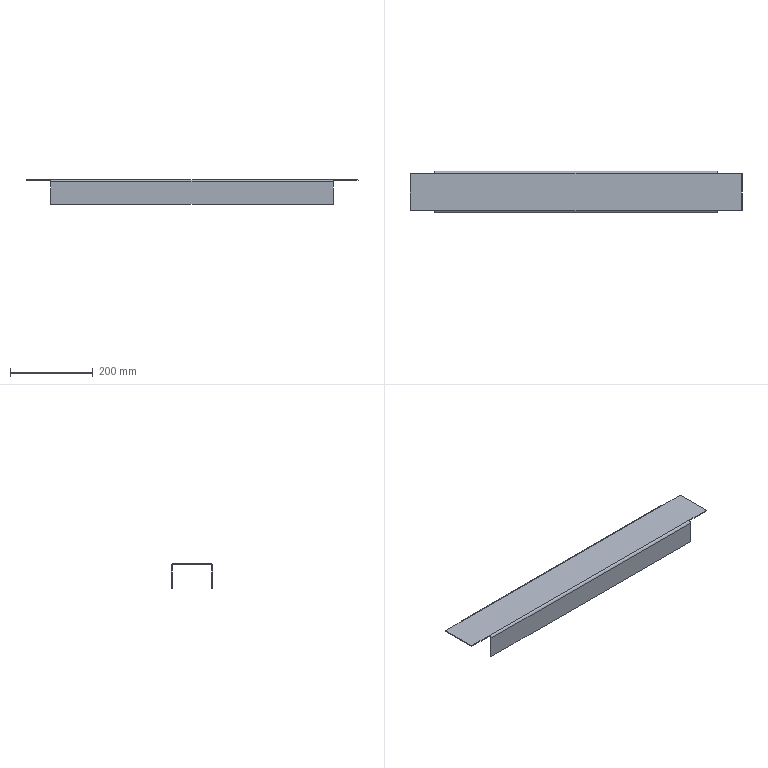Component | SolidWorks | Base-1_BaseFront-Rear-2 | 1 solid | 26 faces | box 800 x 100 x 60 mm | volume 309867 mm3 | plane 22 | cylinder 4 | commonest cylinder face diameters 7 x2 11 x2
STEP:
#1=COLOUR_RGB('',0.7922,0.8196,0.9333);
#2=FILL_AREA_STYLE_COLOUR('',#1);
#3=FILL_AREA_STYLE('',(#2));
#4=SURFACE_STYLE_FILL_AREA(#3);
#5=SURFACE_SIDE_STYLE('',(#4));
#6=SURFACE_STYLE_USAGE(.BOTH.,#5);
#7=PRESENTATION_STYLE_ASSIGNMENT((#6));
#8=CARTESIAN_POINT('',(-16.656,-4.943,13.877));
#9=VERTEX_POINT('',#8);
#10=CARTESIAN_POINT('',(-16.656,-4.943,16.023));
#11=VERTEX_POINT('',#10);
#12=CARTESIAN_POINT('',(-16.656,-4.943,16.239));
#13=DIRECTION('',(-0.,-0.,1.));
#14=VECTOR('',#13,39.37);
#15=LINE('',#12,#14);
#16=EDGE_CURVE('',#9,#11,#15,.T.);
#17=ORIENTED_EDGE('',*,*,#16,.T.);
#18=CARTESIAN_POINT('',(10.116,-4.943,16.023));
#19=VERTEX_POINT('',#18);
#20=CARTESIAN_POINT('',(-19.018,-4.943,16.023));
#21=DIRECTION('',(1.,-0.,0.));
#22=VECTOR('',#21,39.37);
#23=LINE('',#20,#22);
#24=EDGE_CURVE('',#11,#19,#23,.T.);
#25=ORIENTED_EDGE('',*,*,#24,.T.);
#26=CARTESIAN_POINT('',(10.116,-4.943,13.877));
#27=VERTEX_POINT('',#26);
#28=CARTESIAN_POINT('',(10.116,-4.943,16.239));
#29=DIRECTION('',(0.,0.,-1.));
#30=VECTOR('',#29,39.37);
#31=LINE('',#28,#30);
#32=EDGE_CURVE('',#19,#27,#31,.T.);
#33=ORIENTED_EDGE('',*,*,#32,.T.);
#34=CARTESIAN_POINT('',(-19.018,-4.943,13.877));
#35=DIRECTION('',(1.,-0.,0.));
#36=VECTOR('',#35,39.37);
#37=LINE('',#34,#36);
#38=EDGE_CURVE('',#9,#27,#37,.T.);
#39=ORIENTED_EDGE('',*,*,#38,.F.);
#40=EDGE_LOOP('',(#17,#25,#33,#39));
#41=FACE_OUTER_BOUND('',#40,.T.);
#42=CARTESIAN_POINT('',(-19.018,-4.943,16.239));
#43=DIRECTION('',(-0.,-1.,-0.));
#44=DIRECTION('',(-0.,-0.,1.));
#45=AXIS2_PLACEMENT_3D('',#42,#43,#44);
#46=PLANE('',#45);
#47=ADVANCED_FACE('',(#41),#46,.F.);
#48=CARTESIAN_POINT('',(-16.656,-5.021,13.877));
#49=VERTEX_POINT('',#48);
#50=CARTESIAN_POINT('',(10.116,-5.021,13.877));
#51=VERTEX_POINT('',#50);
#52=CARTESIAN_POINT('',(-19.018,-5.021,13.877));
#53=DIRECTION('',(1.,-0.,0.));
#54=VECTOR('',#53,39.37);
#55=LINE('',#52,#54);
#56=EDGE_CURVE('',#49,#51,#55,.T.);
#57=ORIENTED_EDGE('',*,*,#56,.F.);
#58=CARTESIAN_POINT('',(-16.656,-5.021,13.877));
#59=DIRECTION('',(0.,1.,0.));
#60=VECTOR('',#59,39.37);
#61=LINE('',#58,#60);
#62=EDGE_CURVE('',#49,#9,#61,.T.);
#63=ORIENTED_EDGE('',*,*,#62,.T.);
#64=ORIENTED_EDGE('',*,*,#38,.T.);
#65=CARTESIAN_POINT('',(10.116,-5.021,13.877));
#66=DIRECTION('',(0.,1.,0.));
#67=VECTOR('',#66,39.37);
#68=LINE('',#65,#67);
#69=EDGE_CURVE('',#51,#27,#68,.T.);
#70=ORIENTED_EDGE('',*,*,#69,.F.);
#71=EDGE_LOOP('',(#57,#63,#64,#70));
#72=FACE_OUTER_BOUND('',#71,.T.);
#73=CARTESIAN_POINT('',(-19.018,-5.021,13.877));
#74=DIRECTION('',(0.,0.,-1.));
#75=DIRECTION('',(-0.,-1.,-0.));
#76=AXIS2_PLACEMENT_3D('',#73,#74,#75);
#77=PLANE('',#76);
#78=ADVANCED_FACE('',(#72),#77,.T.);
#79=CARTESIAN_POINT('',(-16.656,-5.021,16.023));
#80=VERTEX_POINT('',#79);
#81=CARTESIAN_POINT('',(10.116,-5.021,16.023));
#82=VERTEX_POINT('',#81);
#83=CARTESIAN_POINT('',(-19.018,-5.021,16.023));
#84=DIRECTION('',(1.,-0.,0.));
#85=VECTOR('',#84,39.37);
#86=LINE('',#83,#85);
#87=EDGE_CURVE('',#80,#82,#86,.T.);
#88=ORIENTED_EDGE('',*,*,#87,.F.);
#89=CARTESIAN_POINT('',(-16.656,-5.021,16.239));
#90=DIRECTION('',(-0.,-0.,1.));
#91=VECTOR('',#90,39.37);
#92=LINE('',#89,#91);
#93=EDGE_CURVE('',#49,#80,#92,.T.);
#94=ORIENTED_EDGE('',*,*,#93,.F.);
#95=ORIENTED_EDGE('',*,*,#56,.T.);
#96=CARTESIAN_POINT('',(10.116,-5.021,16.239));
#97=DIRECTION('',(0.,0.,-1.));
#98=VECTOR('',#97,39.37);
#99=LINE('',#96,#98);
#100=EDGE_CURVE('',#82,#51,#99,.T.);
#101=ORIENTED_EDGE('',*,*,#100,.F.);
#102=EDGE_LOOP('',(#88,#94,#95,#101));
#103=FACE_OUTER_BOUND('',#102,.T.);
#104=CARTESIAN_POINT('',(-19.018,-5.021,16.239));
#105=DIRECTION('',(-0.,-1.,-0.));
#106=DIRECTION('',(-0.,-0.,1.));
#107=AXIS2_PLACEMENT_3D('',#104,#105,#106);
#108=PLANE('',#107);
#109=ADVANCED_FACE('',(#103),#108,.T.);
#110=CARTESIAN_POINT('',(-16.656,-5.159,16.16));
#111=VERTEX_POINT('',#110);
#112=CARTESIAN_POINT('',(10.116,-5.159,16.16));
#113=VERTEX_POINT('',#112);
#114=CARTESIAN_POINT('',(-19.018,-5.159,16.16));
#115=DIRECTION('',(1.,-0.,0.));
#116=VECTOR('',#115,39.37);
#117=LINE('',#114,#116);
#118=EDGE_CURVE('',#111,#113,#117,.T.);
#119=ORIENTED_EDGE('',*,*,#118,.F.);
#120=CARTESIAN_POINT('',(-16.656,-5.159,16.023));
#121=DIRECTION('',(1.,-0.,0.));
#122=DIRECTION('',(0.,0.,-1.));
#123=AXIS2_PLACEMENT_3D('',#120,#121,#122);
#124=CIRCLE('',#123,0.1378);
#125=EDGE_CURVE('',#80,#111,#124,.T.);
#126=ORIENTED_EDGE('',*,*,#125,.F.);
#127=ORIENTED_EDGE('',*,*,#87,.T.);
#128=CARTESIAN_POINT('',(10.116,-5.159,16.023));
#129=DIRECTION('',(-1.,0.,-0.));
#130=DIRECTION('',(0.,-1.,0.));
#131=AXIS2_PLACEMENT_3D('',#128,#129,#130);
#132=CIRCLE('',#131,0.1378);
#133=EDGE_CURVE('',#113,#82,#132,.T.);
#134=ORIENTED_EDGE('',*,*,#133,.F.);
#135=EDGE_LOOP('',(#119,#126,#127,#134));
#136=FACE_OUTER_BOUND('',#135,.T.);
#137=CARTESIAN_POINT('',(-19.018,-5.159,16.023));
#138=DIRECTION('',(1.,-0.,0.));
#139=DIRECTION('',(0.,0.,-1.));
#140=AXIS2_PLACEMENT_3D('',#137,#138,#139);
#141=CYLINDRICAL_SURFACE('',#140,0.1378);
#142=ADVANCED_FACE('',(#136),#141,.F.);
#143=CARTESIAN_POINT('',(-16.656,-5.159,16.239));
#144=VERTEX_POINT('',#143);
#145=CARTESIAN_POINT('',(-16.656,-5.159,16.023));
#146=DIRECTION('',(1.,-0.,0.));
#147=DIRECTION('',(0.,0.,-1.));
#148=AXIS2_PLACEMENT_3D('',#145,#146,#147);
#149=CIRCLE('',#148,0.2165);
#150=EDGE_CURVE('',#11,#144,#149,.T.);
#151=ORIENTED_EDGE('',*,*,#150,.T.);
#152=CARTESIAN_POINT('',(10.116,-5.159,16.239));
#153=VERTEX_POINT('',#152);
#154=CARTESIAN_POINT('',(-19.018,-5.159,16.239));
#155=DIRECTION('',(1.,-0.,0.));
#156=VECTOR('',#155,39.37);
#157=LINE('',#154,#156);
#158=EDGE_CURVE('',#144,#153,#157,.T.);
#159=ORIENTED_EDGE('',*,*,#158,.T.);
#160=CARTESIAN_POINT('',(10.116,-5.159,16.023));
#161=DIRECTION('',(-1.,0.,-0.));
#162=DIRECTION('',(0.,0.,-1.));
#163=AXIS2_PLACEMENT_3D('',#160,#161,#162);
#164=CIRCLE('',#163,0.2165);
#165=EDGE_CURVE('',#153,#19,#164,.T.);
#166=ORIENTED_EDGE('',*,*,#165,.T.);
#167=ORIENTED_EDGE('',*,*,#24,.F.);
#168=EDGE_LOOP('',(#151,#159,#166,#167));
#169=FACE_OUTER_BOUND('',#168,.T.);
#170=CARTESIAN_POINT('',(-19.018,-5.159,16.023));
#171=DIRECTION('',(1.,-0.,0.));
#172=DIRECTION('',(0.,0.,-1.));
#173=AXIS2_PLACEMENT_3D('',#170,#171,#172);
#174=CYLINDRICAL_SURFACE('',#173,0.2165);
#175=ADVANCED_FACE('',(#169),#174,.T.);
#176=CARTESIAN_POINT('',(-16.656,-8.663,16.16));
#177=VERTEX_POINT('',#176);
#178=CARTESIAN_POINT('',(10.116,-8.663,16.16));
#179=VERTEX_POINT('',#178);
#180=CARTESIAN_POINT('',(-19.018,-8.663,16.16));
#181=DIRECTION('',(1.,-0.,0.));
#182=VECTOR('',#181,39.37);
#183=LINE('',#180,#182);
#184=EDGE_CURVE('',#177,#179,#183,.T.);
#185=ORIENTED_EDGE('',*,*,#184,.T.);
#186=CARTESIAN_POINT('',(10.116,-8.801,16.023));
#187=VERTEX_POINT('',#186);
#188=CARTESIAN_POINT('',(10.116,-8.663,16.023));
#189=DIRECTION('',(-1.,0.,-0.));
#190=DIRECTION('',(0.,-1.,0.));
#191=AXIS2_PLACEMENT_3D('',#188,#189,#190);
#192=CIRCLE('',#191,0.1378);
#193=EDGE_CURVE('',#187,#179,#192,.T.);
#194=ORIENTED_EDGE('',*,*,#193,.F.);
#195=CARTESIAN_POINT('',(-16.656,-8.801,16.023));
#196=VERTEX_POINT('',#195);
#197=CARTESIAN_POINT('',(-19.018,-8.801,16.023));
#198=DIRECTION('',(1.,-0.,0.));
#199=VECTOR('',#198,39.37);
#200=LINE('',#197,#199);
#201=EDGE_CURVE('',#196,#187,#200,.T.);
#202=ORIENTED_EDGE('',*,*,#201,.F.);
#203=CARTESIAN_POINT('',(-16.656,-8.663,16.023));
#204=DIRECTION('',(1.,-0.,0.));
#205=DIRECTION('',(0.,0.,-1.));
#206=AXIS2_PLACEMENT_3D('',#203,#204,#205);
#207=CIRCLE('',#206,0.1378);
#208=EDGE_CURVE('',#177,#196,#207,.T.);
#209=ORIENTED_EDGE('',*,*,#208,.F.);
#210=EDGE_LOOP('',(#185,#194,#202,#209));
#211=FACE_OUTER_BOUND('',#210,.T.);
#212=CARTESIAN_POINT('',(-19.018,-8.663,16.023));
#213=DIRECTION('',(1.,-0.,0.));
#214=DIRECTION('',(0.,0.,-1.));
#215=AXIS2_PLACEMENT_3D('',#212,#213,#214);
#216=CYLINDRICAL_SURFACE('',#215,0.1378);
#217=ADVANCED_FACE('',(#211),#216,.F.);
#218=ORIENTED_EDGE('',*,*,#201,.T.);
#219=CARTESIAN_POINT('',(10.116,-8.801,13.877));
#220=VERTEX_POINT('',#219);
#221=CARTESIAN_POINT('',(10.116,-8.801,13.877));
#222=DIRECTION('',(-0.,-0.,1.));
#223=VECTOR('',#222,39.37);
#224=LINE('',#221,#223);
#225=EDGE_CURVE('',#220,#187,#224,.T.);
#226=ORIENTED_EDGE('',*,*,#225,.F.);
#227=CARTESIAN_POINT('',(-16.656,-8.801,13.877));
#228=VERTEX_POINT('',#227);
#229=CARTESIAN_POINT('',(-19.018,-8.801,13.877));
#230=DIRECTION('',(1.,-0.,0.));
#231=VECTOR('',#230,39.37);
#232=LINE('',#229,#231);
#233=EDGE_CURVE('',#228,#220,#232,.T.);
#234=ORIENTED_EDGE('',*,*,#233,.F.);
#235=CARTESIAN_POINT('',(-16.656,-8.801,13.877));
#236=DIRECTION('',(0.,0.,-1.));
#237=VECTOR('',#236,39.37);
#238=LINE('',#235,#237);
#239=EDGE_CURVE('',#196,#228,#238,.T.);
#240=ORIENTED_EDGE('',*,*,#239,.F.);
#241=EDGE_LOOP('',(#218,#226,#234,#240));
#242=FACE_OUTER_BOUND('',#241,.T.);
#243=CARTESIAN_POINT('',(-19.018,-8.801,13.877));
#244=DIRECTION('',(0.,1.,0.));
#245=DIRECTION('',(0.,0.,-1.));
#246=AXIS2_PLACEMENT_3D('',#243,#244,#245);
#247=PLANE('',#246);
#248=ADVANCED_FACE('',(#242),#247,.T.);
#249=ORIENTED_EDGE('',*,*,#233,.T.);
#250=CARTESIAN_POINT('',(10.116,-8.88,13.877));
#251=VERTEX_POINT('',#250);
#252=CARTESIAN_POINT('',(10.116,-8.801,13.877));
#253=DIRECTION('',(-0.,-1.,-0.));
#254=VECTOR('',#253,39.37);
#255=LINE('',#252,#254);
#256=EDGE_CURVE('',#220,#251,#255,.T.);
#257=ORIENTED_EDGE('',*,*,#256,.T.);
#258=CARTESIAN_POINT('',(-16.656,-8.88,13.877));
#259=VERTEX_POINT('',#258);
#260=CARTESIAN_POINT('',(-19.018,-8.88,13.877));
#261=DIRECTION('',(1.,-0.,0.));
#262=VECTOR('',#261,39.37);
#263=LINE('',#260,#262);
#264=EDGE_CURVE('',#259,#251,#263,.T.);
#265=ORIENTED_EDGE('',*,*,#264,.F.);
#266=CARTESIAN_POINT('',(-16.656,-8.88,13.877));
#267=DIRECTION('',(0.,1.,0.));
#268=VECTOR('',#267,39.37);
#269=LINE('',#266,#268);
#270=EDGE_CURVE('',#259,#228,#269,.T.);
#271=ORIENTED_EDGE('',*,*,#270,.T.);
#272=EDGE_LOOP('',(#249,#257,#265,#271));
#273=FACE_OUTER_BOUND('',#272,.T.);
#274=CARTESIAN_POINT('',(-19.018,-8.88,13.877));
#275=DIRECTION('',(0.,0.,-1.));
#276=DIRECTION('',(-0.,-1.,-0.));
#277=AXIS2_PLACEMENT_3D('',#274,#275,#276);
#278=PLANE('',#277);
#279=ADVANCED_FACE('',(#273),#278,.T.);
#280=CARTESIAN_POINT('',(10.116,-8.88,16.023));
#281=VERTEX_POINT('',#280);
#282=CARTESIAN_POINT('',(10.116,-8.88,13.877));
#283=DIRECTION('',(-0.,-0.,1.));
#284=VECTOR('',#283,39.37);
#285=LINE('',#282,#284);
#286=EDGE_CURVE('',#251,#281,#285,.T.);
#287=ORIENTED_EDGE('',*,*,#286,.T.);
#288=CARTESIAN_POINT('',(-16.656,-8.88,16.023));
#289=VERTEX_POINT('',#288);
#290=CARTESIAN_POINT('',(-19.018,-8.88,16.023));
#291=DIRECTION('',(1.,-0.,0.));
#292=VECTOR('',#291,39.37);
#293=LINE('',#290,#292);
#294=EDGE_CURVE('',#289,#281,#293,.T.);
#295=ORIENTED_EDGE('',*,*,#294,.F.);
#296=CARTESIAN_POINT('',(-16.656,-8.88,20.752));
#297=DIRECTION('',(0.,0.,-1.));
#298=VECTOR('',#297,39.37);
#299=LINE('',#296,#298);
#300=EDGE_CURVE('',#289,#259,#299,.T.);
#301=ORIENTED_EDGE('',*,*,#300,.T.);
#302=ORIENTED_EDGE('',*,*,#264,.T.);
#303=EDGE_LOOP('',(#287,#295,#301,#302));
#304=FACE_OUTER_BOUND('',#303,.T.);
#305=CARTESIAN_POINT('',(-19.018,-8.88,13.877));
#306=DIRECTION('',(0.,1.,0.));
#307=DIRECTION('',(0.,0.,-1.));
#308=AXIS2_PLACEMENT_3D('',#305,#306,#307);
#309=PLANE('',#308);
#310=ADVANCED_FACE('',(#304),#309,.F.);
#311=CARTESIAN_POINT('',(10.116,-8.663,16.239));
#312=VERTEX_POINT('',#311);
#313=CARTESIAN_POINT('',(10.116,-8.663,16.023));
#314=DIRECTION('',(-1.,0.,-0.));
#315=DIRECTION('',(0.,0.,-1.));
#316=AXIS2_PLACEMENT_3D('',#313,#314,#315);
#317=CIRCLE('',#316,0.2165);
#318=EDGE_CURVE('',#281,#312,#317,.T.);
#319=ORIENTED_EDGE('',*,*,#318,.T.);
#320=CARTESIAN_POINT('',(-16.656,-8.663,16.239));
#321=VERTEX_POINT('',#320);
#322=CARTESIAN_POINT('',(-19.018,-8.663,16.239));
#323=DIRECTION('',(1.,-0.,0.));
#324=VECTOR('',#323,39.37);
#325=LINE('',#322,#324);
#326=EDGE_CURVE('',#321,#312,#325,.T.);
#327=ORIENTED_EDGE('',*,*,#326,.F.);
#328=CARTESIAN_POINT('',(-16.656,-8.663,16.023));
#329=DIRECTION('',(1.,-0.,0.));
#330=DIRECTION('',(0.,0.,-1.));
#331=AXIS2_PLACEMENT_3D('',#328,#329,#330);
#332=CIRCLE('',#331,0.2165);
#333=EDGE_CURVE('',#321,#289,#332,.T.);
#334=ORIENTED_EDGE('',*,*,#333,.T.);
#335=ORIENTED_EDGE('',*,*,#294,.T.);
#336=EDGE_LOOP('',(#319,#327,#334,#335));
#337=FACE_OUTER_BOUND('',#336,.T.);
#338=CARTESIAN_POINT('',(-19.018,-8.663,16.023));
#339=DIRECTION('',(1.,-0.,0.));
#340=DIRECTION('',(0.,0.,-1.));
#341=AXIS2_PLACEMENT_3D('',#338,#339,#340);
#342=CYLINDRICAL_SURFACE('',#341,0.2165);
#343=ADVANCED_FACE('',(#337),#342,.T.);
#344=CARTESIAN_POINT('',(12.478,-8.663,16.239));
#345=VERTEX_POINT('',#344);
#346=CARTESIAN_POINT('',(12.478,-5.159,16.239));
#347=VERTEX_POINT('',#346);
#348=CARTESIAN_POINT('',(12.478,-8.88,16.239));
#349=DIRECTION('',(0.,1.,0.));
#350=VECTOR('',#349,39.37);
#351=LINE('',#348,#350);
#352=EDGE_CURVE('',#345,#347,#351,.T.);
#353=ORIENTED_EDGE('',*,*,#352,.F.);
#354=CARTESIAN_POINT('',(12.478,-8.663,16.16));
#355=VERTEX_POINT('',#354);
#356=CARTESIAN_POINT('',(12.478,-8.663,16.239));
#357=DIRECTION('',(0.,0.,-1.));
#358=VECTOR('',#357,39.37);
#359=LINE('',#356,#358);
#360=EDGE_CURVE('',#345,#355,#359,.T.);
#361=ORIENTED_EDGE('',*,*,#360,.T.);
#362=CARTESIAN_POINT('',(12.478,-5.159,16.16));
#363=VERTEX_POINT('',#362);
#364=CARTESIAN_POINT('',(12.478,-8.88,16.16));
#365=DIRECTION('',(0.,1.,0.));
#366=VECTOR('',#365,39.37);
#367=LINE('',#364,#366);
#368=EDGE_CURVE('',#355,#363,#367,.T.);
#369=ORIENTED_EDGE('',*,*,#368,.T.);
#370=CARTESIAN_POINT('',(12.478,-5.159,16.16));
#371=DIRECTION('',(-0.,-0.,1.));
#372=VECTOR('',#371,39.37);
#373=LINE('',#370,#372);
#374=EDGE_CURVE('',#363,#347,#373,.T.);
#375=ORIENTED_EDGE('',*,*,#374,.T.);
#376=EDGE_LOOP('',(#353,#361,#369,#375));
#377=FACE_OUTER_BOUND('',#376,.T.);
#378=CARTESIAN_POINT('',(12.478,-8.801,16.023));
#379=DIRECTION('',(1.,-0.,0.));
#380=DIRECTION('',(0.,0.,-1.));
#381=AXIS2_PLACEMENT_3D('',#378,#379,#380);
#382=PLANE('',#381);
#383=ADVANCED_FACE('',(#377),#382,.T.);
#384=CARTESIAN_POINT('',(-19.018,-8.663,16.239));
#385=VERTEX_POINT('',#384);
#386=CARTESIAN_POINT('',(-19.018,-5.159,16.239));
#387=VERTEX_POINT('',#386);
#388=CARTESIAN_POINT('',(-19.018,-8.88,16.239));
#389=DIRECTION('',(0.,1.,0.));
#390=VECTOR('',#389,39.37);
#391=LINE('',#388,#390);
#392=EDGE_CURVE('',#385,#387,#391,.T.);
#393=ORIENTED_EDGE('',*,*,#392,.T.);
#394=CARTESIAN_POINT('',(-19.018,-5.159,16.16));
#395=VERTEX_POINT('',#394);
#396=CARTESIAN_POINT('',(-19.018,-5.159,16.239));
#397=DIRECTION('',(0.,0.,-1.));
#398=VECTOR('',#397,39.37);
#399=LINE('',#396,#398);
#400=EDGE_CURVE('',#387,#395,#399,.T.);
#401=ORIENTED_EDGE('',*,*,#400,.T.);
#402=CARTESIAN_POINT('',(-19.018,-8.663,16.16));
#403=VERTEX_POINT('',#402);
#404=CARTESIAN_POINT('',(-19.018,-8.88,16.16));
#405=DIRECTION('',(0.,1.,0.));
#406=VECTOR('',#405,39.37);
#407=LINE('',#404,#406);
#408=EDGE_CURVE('',#403,#395,#407,.T.);
#409=ORIENTED_EDGE('',*,*,#408,.F.);
#410=CARTESIAN_POINT('',(-19.018,-8.663,16.16));
#411=DIRECTION('',(-0.,-0.,1.));
#412=VECTOR('',#411,39.37);
#413=LINE('',#410,#412);
#414=EDGE_CURVE('',#403,#385,#413,.T.);
#415=ORIENTED_EDGE('',*,*,#414,.T.);
#416=EDGE_LOOP('',(#393,#401,#409,#415));
#417=FACE_OUTER_BOUND('',#416,.T.);
#418=CARTESIAN_POINT('',(-19.018,-5.021,16.023));
#419=DIRECTION('',(-1.,0.,-0.));
#420=DIRECTION('',(-0.,-0.,1.));
#421=AXIS2_PLACEMENT_3D('',#418,#419,#420);
#422=PLANE('',#421);
#423=ADVANCED_FACE('',(#417),#422,.T.);
#424=ORIENTED_EDGE('',*,*,#368,.F.);
#425=CARTESIAN_POINT('',(-19.018,-8.663,16.16));
#426=DIRECTION('',(1.,-0.,0.));
#427=VECTOR('',#426,39.37);
#428=LINE('',#425,#427);
#429=EDGE_CURVE('',#179,#355,#428,.T.);
#430=ORIENTED_EDGE('',*,*,#429,.F.);
#431=ORIENTED_EDGE('',*,*,#184,.F.);
#432=CARTESIAN_POINT('',(-19.018,-8.663,16.16));
#433=DIRECTION('',(1.,-0.,0.));
#434=VECTOR('',#433,39.37);
#435=LINE('',#432,#434);
#436=EDGE_CURVE('',#403,#177,#435,.T.);
#437=ORIENTED_EDGE('',*,*,#436,.F.);
#438=ORIENTED_EDGE('',*,*,#408,.T.);
#439=CARTESIAN_POINT('',(-19.018,-5.159,16.16));
#440=DIRECTION('',(1.,-0.,0.));
#441=VECTOR('',#440,39.37);
#442=LINE('',#439,#441);
#443=EDGE_CURVE('',#395,#111,#442,.T.);
#444=ORIENTED_EDGE('',*,*,#443,.T.);
#445=ORIENTED_EDGE('',*,*,#118,.T.);
#446=CARTESIAN_POINT('',(-19.018,-5.159,16.16));
#447=DIRECTION('',(1.,-0.,0.));
#448=VECTOR('',#447,39.37);
#449=LINE('',#446,#448);
#450=EDGE_CURVE('',#113,#363,#449,.T.);
#451=ORIENTED_EDGE('',*,*,#450,.T.);
#452=EDGE_LOOP('',(#424,#430,#431,#437,#438,#444,#445,#451));
#453=FACE_OUTER_BOUND('',#452,.T.);
#454=CARTESIAN_POINT('',(-19.018,-8.88,16.16));
#455=DIRECTION('',(0.,0.,-1.));
#456=DIRECTION('',(-0.,-1.,-0.));
#457=AXIS2_PLACEMENT_3D('',#454,#455,#456);
#458=PLANE('',#457);
#459=ADVANCED_FACE('',(#453),#458,.T.);
#460=ORIENTED_EDGE('',*,*,#352,.T.);
#461=CARTESIAN_POINT('',(-19.018,-5.159,16.239));
#462=DIRECTION('',(1.,-0.,0.));
#463=VECTOR('',#462,39.37);
#464=LINE('',#461,#463);
#465=EDGE_CURVE('',#153,#347,#464,.T.);
#466=ORIENTED_EDGE('',*,*,#465,.F.);
#467=ORIENTED_EDGE('',*,*,#158,.F.);
#468=CARTESIAN_POINT('',(-19.018,-5.159,16.239));
#469=DIRECTION('',(1.,-0.,0.));
#470=VECTOR('',#469,39.37);
#471=LINE('',#468,#470);
#472=EDGE_CURVE('',#387,#144,#471,.T.);
#473=ORIENTED_EDGE('',*,*,#472,.F.);
#474=ORIENTED_EDGE('',*,*,#392,.F.);
#475=CARTESIAN_POINT('',(-19.018,-8.663,16.239));
#476=DIRECTION('',(1.,-0.,0.));
#477=VECTOR('',#476,39.37);
#478=LINE('',#475,#477);
#479=EDGE_CURVE('',#385,#321,#478,.T.);
#480=ORIENTED_EDGE('',*,*,#479,.T.);
#481=ORIENTED_EDGE('',*,*,#326,.T.);
#482=CARTESIAN_POINT('',(-19.018,-8.663,16.239));
#483=DIRECTION('',(1.,-0.,0.));
#484=VECTOR('',#483,39.37);
#485=LINE('',#482,#484);
#486=EDGE_CURVE('',#312,#345,#485,.T.);
#487=ORIENTED_EDGE('',*,*,#486,.T.);
#488=EDGE_LOOP('',(#460,#466,#467,#473,#474,#480,#481,#487));
#489=FACE_OUTER_BOUND('',#488,.T.);
#490=CARTESIAN_POINT('',(-19.018,-8.88,16.239));
#491=DIRECTION('',(0.,0.,-1.));
#492=DIRECTION('',(-0.,-1.,-0.));
#493=AXIS2_PLACEMENT_3D('',#490,#491,#492);
#494=PLANE('',#493);
#495=ADVANCED_FACE('',(#489),#494,.F.);
#496=ORIENTED_EDGE('',*,*,#270,.F.);
#497=ORIENTED_EDGE('',*,*,#300,.F.);
#498=CARTESIAN_POINT('',(-16.656,-8.88,16.023));
#499=DIRECTION('',(0.,1.,0.));
#500=VECTOR('',#499,39.37);
#501=LINE('',#498,#500);
#502=EDGE_CURVE('',#289,#196,#501,.T.);
#503=ORIENTED_EDGE('',*,*,#502,.T.);
#504=ORIENTED_EDGE('',*,*,#239,.T.);
#505=EDGE_LOOP('',(#496,#497,#503,#504));
#506=FACE_OUTER_BOUND('',#505,.T.);
#507=CARTESIAN_POINT('',(-16.656,-8.88,20.752));
#508=DIRECTION('',(1.,-0.,0.));
#509=DIRECTION('',(0.,0.,-1.));
#510=AXIS2_PLACEMENT_3D('',#507,#508,#509);
#511=PLANE('',#510);
#512=ADVANCED_FACE('',(#506),#511,.F.);
#513=ORIENTED_EDGE('',*,*,#414,.F.);
#514=ORIENTED_EDGE('',*,*,#436,.T.);
#515=CARTESIAN_POINT('',(-16.656,-8.663,16.16));
#516=DIRECTION('',(-0.,-0.,1.));
#517=VECTOR('',#516,39.37);
#518=LINE('',#515,#517);
#519=EDGE_CURVE('',#177,#321,#518,.T.);
#520=ORIENTED_EDGE('',*,*,#519,.T.);
#521=ORIENTED_EDGE('',*,*,#479,.F.);
#522=EDGE_LOOP('',(#513,#514,#520,#521));
#523=FACE_OUTER_BOUND('',#522,.T.);
#524=CARTESIAN_POINT('',(-17.837,-8.663,16.16));
#525=DIRECTION('',(-0.,-1.,-0.));
#526=DIRECTION('',(1.,-0.,0.));
#527=AXIS2_PLACEMENT_3D('',#524,#525,#526);
#528=PLANE('',#527);
#529=ADVANCED_FACE('',(#523),#528,.T.);
#530=ORIENTED_EDGE('',*,*,#502,.F.);
#531=ORIENTED_EDGE('',*,*,#333,.F.);
#532=ORIENTED_EDGE('',*,*,#519,.F.);
#533=ORIENTED_EDGE('',*,*,#208,.T.);
#534=EDGE_LOOP('',(#530,#531,#532,#533));
#535=FACE_OUTER_BOUND('',#534,.T.);
#536=CARTESIAN_POINT('',(-16.656,-8.663,16.023));
#537=DIRECTION('',(-1.,0.,-0.));
#538=DIRECTION('',(-0.,-0.,1.));
#539=AXIS2_PLACEMENT_3D('',#536,#537,#538);
#540=PLANE('',#539);
#541=ADVANCED_FACE('',(#535),#540,.T.);
#542=ORIENTED_EDGE('',*,*,#225,.T.);
#543=CARTESIAN_POINT('',(10.116,-8.801,16.023));
#544=DIRECTION('',(-0.,-1.,-0.));
#545=VECTOR('',#544,39.37);
#546=LINE('',#543,#545);
#547=EDGE_CURVE('',#187,#281,#546,.T.);
#548=ORIENTED_EDGE('',*,*,#547,.T.);
#549=ORIENTED_EDGE('',*,*,#286,.F.);
#550=ORIENTED_EDGE('',*,*,#256,.F.);
#551=EDGE_LOOP('',(#542,#548,#549,#550));
#552=FACE_OUTER_BOUND('',#551,.T.);
#553=CARTESIAN_POINT('',(10.116,-8.801,13.877));
#554=DIRECTION('',(-1.,0.,-0.));
#555=DIRECTION('',(-0.,-0.,1.));
#556=AXIS2_PLACEMENT_3D('',#553,#554,#555);
#557=PLANE('',#556);
#558=ADVANCED_FACE('',(#552),#557,.F.);
#559=CARTESIAN_POINT('',(10.116,-8.663,16.16));
#560=DIRECTION('',(-0.,-0.,1.));
#561=VECTOR('',#560,39.37);
#562=LINE('',#559,#561);
#563=EDGE_CURVE('',#179,#312,#562,.T.);
#564=ORIENTED_EDGE('',*,*,#563,.F.);
#565=ORIENTED_EDGE('',*,*,#429,.T.);
#566=ORIENTED_EDGE('',*,*,#360,.F.);
#567=ORIENTED_EDGE('',*,*,#486,.F.);
#568=EDGE_LOOP('',(#564,#565,#566,#567));
#569=FACE_OUTER_BOUND('',#568,.T.);
#570=CARTESIAN_POINT('',(11.297,-8.663,16.16));
#571=DIRECTION('',(-0.,-1.,-0.));
#572=DIRECTION('',(1.,-0.,0.));
#573=AXIS2_PLACEMENT_3D('',#570,#571,#572);
#574=PLANE('',#573);
#575=ADVANCED_FACE('',(#569),#574,.T.);
#576=ORIENTED_EDGE('',*,*,#318,.F.);
#577=ORIENTED_EDGE('',*,*,#547,.F.);
#578=ORIENTED_EDGE('',*,*,#193,.T.);
#579=ORIENTED_EDGE('',*,*,#563,.T.);
#580=EDGE_LOOP('',(#576,#577,#578,#579));
#581=FACE_OUTER_BOUND('',#580,.T.);
#582=CARTESIAN_POINT('',(10.116,-8.663,16.023));
#583=DIRECTION('',(1.,-0.,0.));
#584=DIRECTION('',(0.,1.,0.));
#585=AXIS2_PLACEMENT_3D('',#582,#583,#584);
#586=PLANE('',#585);
#587=ADVANCED_FACE('',(#581),#586,.T.);
#588=ORIENTED_EDGE('',*,*,#100,.T.);
#589=ORIENTED_EDGE('',*,*,#69,.T.);
#590=ORIENTED_EDGE('',*,*,#32,.F.);
#591=CARTESIAN_POINT('',(10.116,-5.021,16.023));
#592=DIRECTION('',(0.,1.,0.));
#593=VECTOR('',#592,39.37);
#594=LINE('',#591,#593);
#595=EDGE_CURVE('',#82,#19,#594,.T.);
#596=ORIENTED_EDGE('',*,*,#595,.F.);
#597=EDGE_LOOP('',(#588,#589,#590,#596));
#598=FACE_OUTER_BOUND('',#597,.T.);
#599=CARTESIAN_POINT('',(10.116,-5.021,16.239));
#600=DIRECTION('',(-1.,0.,-0.));
#601=DIRECTION('',(0.,0.,-1.));
#602=AXIS2_PLACEMENT_3D('',#599,#600,#601);
#603=PLANE('',#602);
#604=ADVANCED_FACE('',(#598),#603,.F.);
#605=ORIENTED_EDGE('',*,*,#374,.F.);
#606=ORIENTED_EDGE('',*,*,#450,.F.);
#607=CARTESIAN_POINT('',(10.116,-5.159,16.16));
#608=DIRECTION('',(-0.,-0.,1.));
#609=VECTOR('',#608,39.37);
#610=LINE('',#607,#609);
#611=EDGE_CURVE('',#113,#153,#610,.T.);
#612=ORIENTED_EDGE('',*,*,#611,.T.);
#613=ORIENTED_EDGE('',*,*,#465,.T.);
#614=EDGE_LOOP('',(#605,#606,#612,#613));
#615=FACE_OUTER_BOUND('',#614,.T.);
#616=CARTESIAN_POINT('',(11.297,-5.159,16.16));
#617=DIRECTION('',(-0.,-1.,-0.));
#618=DIRECTION('',(1.,-0.,0.));
#619=AXIS2_PLACEMENT_3D('',#616,#617,#618);
#620=PLANE('',#619);
#621=ADVANCED_FACE('',(#615),#620,.F.);
#622=ORIENTED_EDGE('',*,*,#595,.T.);
#623=ORIENTED_EDGE('',*,*,#165,.F.);
#624=ORIENTED_EDGE('',*,*,#611,.F.);
#625=ORIENTED_EDGE('',*,*,#133,.T.);
#626=EDGE_LOOP('',(#622,#623,#624,#625));
#627=FACE_OUTER_BOUND('',#626,.T.);
#628=CARTESIAN_POINT('',(10.116,-5.159,16.023));
#629=DIRECTION('',(1.,-0.,0.));
#630=DIRECTION('',(0.,1.,0.));
#631=AXIS2_PLACEMENT_3D('',#628,#629,#630);
#632=PLANE('',#631);
#633=ADVANCED_FACE('',(#627),#632,.T.);
#634=ORIENTED_EDGE('',*,*,#93,.T.);
#635=CARTESIAN_POINT('',(-16.656,-5.021,16.023));
#636=DIRECTION('',(0.,1.,0.));
#637=VECTOR('',#636,39.37);
#638=LINE('',#635,#637);
#639=EDGE_CURVE('',#80,#11,#638,.T.);
#640=ORIENTED_EDGE('',*,*,#639,.T.);
#641=ORIENTED_EDGE('',*,*,#16,.F.);
#642=ORIENTED_EDGE('',*,*,#62,.F.);
#643=EDGE_LOOP('',(#634,#640,#641,#642));
#644=FACE_OUTER_BOUND('',#643,.T.);
#645=CARTESIAN_POINT('',(-16.656,-5.021,16.239));
#646=DIRECTION('',(1.,-0.,0.));
#647=DIRECTION('',(-0.,-0.,1.));
#648=AXIS2_PLACEMENT_3D('',#645,#646,#647);
#649=PLANE('',#648);
#650=ADVANCED_FACE('',(#644),#649,.F.);
#651=ORIENTED_EDGE('',*,*,#150,.F.);
#652=ORIENTED_EDGE('',*,*,#639,.F.);
#653=ORIENTED_EDGE('',*,*,#125,.T.);
#654=CARTESIAN_POINT('',(-16.656,-5.159,16.16));
#655=DIRECTION('',(-0.,-0.,1.));
#656=VECTOR('',#655,39.37);
#657=LINE('',#654,#656);
#658=EDGE_CURVE('',#111,#144,#657,.T.);
#659=ORIENTED_EDGE('',*,*,#658,.T.);
#660=EDGE_LOOP('',(#651,#652,#653,#659));
#661=FACE_OUTER_BOUND('',#660,.T.);
#662=CARTESIAN_POINT('',(-16.656,-5.159,16.023));
#663=DIRECTION('',(-1.,0.,-0.));
#664=DIRECTION('',(-0.,-0.,1.));
#665=AXIS2_PLACEMENT_3D('',#662,#663,#664);
#666=PLANE('',#665);
#667=ADVANCED_FACE('',(#661),#666,.T.);
#668=ORIENTED_EDGE('',*,*,#658,.F.);
#669=ORIENTED_EDGE('',*,*,#443,.F.);
#670=ORIENTED_EDGE('',*,*,#400,.F.);
#671=ORIENTED_EDGE('',*,*,#472,.T.);
#672=EDGE_LOOP('',(#668,#669,#670,#671));
#673=FACE_OUTER_BOUND('',#672,.T.);
#674=CARTESIAN_POINT('',(-17.837,-5.159,16.16));
#675=DIRECTION('',(-0.,-1.,-0.));
#676=DIRECTION('',(1.,-0.,0.));
#677=AXIS2_PLACEMENT_3D('',#674,#675,#676);
#678=PLANE('',#677);
#679=ADVANCED_FACE('',(#673),#678,.F.);
#680=CLOSED_SHELL('',(#47,#78,#109,#142,#175,#217,#248,#279,#310,#343,#383,#423,#459,#495,#512,#529,#541,#558,#575,#587,#604,#621,#633,#650,#667,#679));
#681=MANIFOLD_SOLID_BREP('',#680);
#682=STYLED_ITEM('',(#7),#681);
#683=(LENGTH_UNIT()NAMED_UNIT(*)SI_UNIT($,.METRE.));
#684=LENGTH_MEASURE_WITH_UNIT(LENGTH_MEASURE(0.0254),#683);
#685=DIMENSIONAL_EXPONENTS(1.,0.,0.,0.,0.,0.,0.);
#686=(CONVERSION_BASED_UNIT('',#684)LENGTH_UNIT()NAMED_UNIT(#685));
#687=UNCERTAINTY_MEASURE_WITH_UNIT(LENGTH_MEASURE(0.00001),#686,'','');
#688=(NAMED_UNIT(*)PLANE_ANGLE_UNIT()SI_UNIT($,.RADIAN.));
#689=(NAMED_UNIT(*)SI_UNIT($,.STERADIAN.)SOLID_ANGLE_UNIT());
#690=(GEOMETRIC_REPRESENTATION_CONTEXT(3)GLOBAL_UNCERTAINTY_ASSIGNED_CONTEXT((#687))GLOBAL_UNIT_ASSIGNED_CONTEXT((#686,#688,#689))REPRESENTATION_CONTEXT('',''));
#691=MECHANICAL_DESIGN_GEOMETRIC_PRESENTATION_REPRESENTATION('',(#682),#690);
#692=PRESENTATION_LAYER_ASSIGNMENT('','',(#682));
#693=CARTESIAN_POINT('',(0.,0.,0.));
#694=DIRECTION('',(0.,0.,1.));
#695=DIRECTION('',(1.,0.,0.));
#696=AXIS2_PLACEMENT_3D('',#693,#694,#695);
#697=(LENGTH_UNIT()NAMED_UNIT(*)SI_UNIT($,.METRE.));
#698=LENGTH_MEASURE_WITH_UNIT(LENGTH_MEASURE(0.0254),#697);
#699=DIMENSIONAL_EXPONENTS(1.,0.,0.,0.,0.,0.,0.);
#700=(CONVERSION_BASED_UNIT('',#698)LENGTH_UNIT()NAMED_UNIT(#699));
#701=UNCERTAINTY_MEASURE_WITH_UNIT(LENGTH_MEASURE(0.00001),#700,'','');
#702=(NAMED_UNIT(*)PLANE_ANGLE_UNIT()SI_UNIT($,.RADIAN.));
#703=(NAMED_UNIT(*)SI_UNIT($,.STERADIAN.)SOLID_ANGLE_UNIT());
#704=(GEOMETRIC_REPRESENTATION_CONTEXT(3)GLOBAL_UNCERTAINTY_ASSIGNED_CONTEXT((#701))GLOBAL_UNIT_ASSIGNED_CONTEXT((#700,#702,#703))REPRESENTATION_CONTEXT('',''));
#705=ADVANCED_BREP_SHAPE_REPRESENTATION('',(#681,#696),#704);